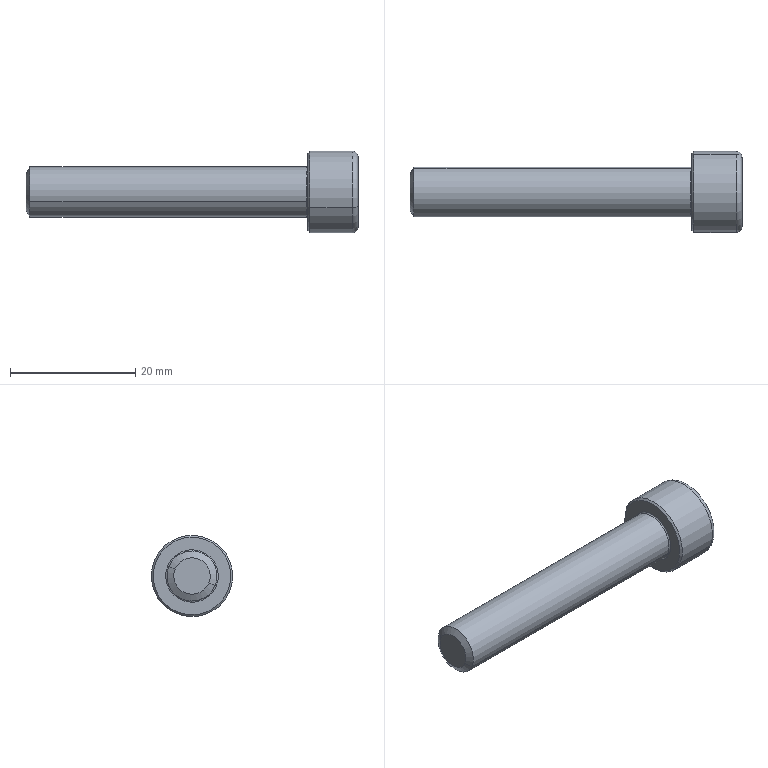Component | SolidWorks | M8_45_T70.1-1 | 1 solid | 28 faces | box 53 x 13 x 13 mm | volume 3185 mm3 | cone 10 | plane 10 | torus 4 | cylinder 4 | commonest cylinder face diameters 13 x2 8 x2 | material Plain Carbon Steel
STEP:
#1=COLOUR_RGB('',0.7922,0.8196,0.9333);
#2=FILL_AREA_STYLE_COLOUR('',#1);
#3=FILL_AREA_STYLE('',(#2));
#4=SURFACE_STYLE_FILL_AREA(#3);
#5=SURFACE_SIDE_STYLE('',(#4));
#6=SURFACE_STYLE_USAGE(.BOTH.,#5);
#7=PRESENTATION_STYLE_ASSIGNMENT((#6));
#8=CARTESIAN_POINT('',(2.524,1.896,1.764));
#9=VERTEX_POINT('',#8);
#10=CARTESIAN_POINT('',(2.524,1.445,1.577));
#11=VERTEX_POINT('',#10);
#12=CARTESIAN_POINT('',(2.524,1.67,1.67));
#13=DIRECTION('',(-1.,0.,-0.));
#14=DIRECTION('',(0.,-0.9242,-0.3818));
#15=AXIS2_PLACEMENT_3D('',#12,#13,#14);
#16=CIRCLE('',#15,0.2441);
#17=EDGE_CURVE('',#9,#11,#16,.T.);
#18=ORIENTED_EDGE('',*,*,#17,.F.);
#19=CARTESIAN_POINT('',(2.535,1.907,1.768));
#20=VERTEX_POINT('',#19);
#21=CARTESIAN_POINT('',(2.535,1.907,1.768));
#22=DIRECTION('',(0.7071,0.6535,0.27));
#23=VECTOR('',#22,39.37);
#24=LINE('',#21,#23);
#25=EDGE_CURVE('',#9,#20,#24,.T.);
#26=ORIENTED_EDGE('',*,*,#25,.T.);
#27=CARTESIAN_POINT('',(2.535,1.434,1.573));
#28=VERTEX_POINT('',#27);
#29=CARTESIAN_POINT('',(2.535,1.67,1.67));
#30=DIRECTION('',(1.,0.,0.));
#31=DIRECTION('',(0.,-0.9242,-0.3818));
#32=AXIS2_PLACEMENT_3D('',#29,#30,#31);
#33=CIRCLE('',#32,0.2559);
#34=EDGE_CURVE('',#28,#20,#33,.T.);
#35=ORIENTED_EDGE('',*,*,#34,.F.);
#36=CARTESIAN_POINT('',(2.535,1.434,1.573));
#37=DIRECTION('',(0.7071,-0.6535,-0.27));
#38=VECTOR('',#37,39.37);
#39=LINE('',#36,#38);
#40=EDGE_CURVE('',#11,#28,#39,.T.);
#41=ORIENTED_EDGE('',*,*,#40,.F.);
#42=EDGE_LOOP('',(#18,#26,#35,#41));
#43=FACE_OUTER_BOUND('',#42,.T.);
#44=CARTESIAN_POINT('',(2.535,1.67,1.67));
#45=DIRECTION('',(1.,0.,0.));
#46=DIRECTION('',(0.,-0.9242,-0.3818));
#47=AXIS2_PLACEMENT_3D('',#44,#45,#46);
#48=CONICAL_SURFACE('',#47,0.2559,0.7854);
#49=ADVANCED_FACE('',(#43),#48,.T.);
#50=CARTESIAN_POINT('',(2.839,1.467,1.586));
#51=VERTEX_POINT('',#50);
#52=CARTESIAN_POINT('',(2.839,1.874,1.755));
#53=VERTEX_POINT('',#52);
#54=CARTESIAN_POINT('',(2.839,1.67,1.67));
#55=DIRECTION('',(1.,0.,0.));
#56=DIRECTION('',(0.,0.9242,0.3818));
#57=AXIS2_PLACEMENT_3D('',#54,#55,#56);
#58=CIRCLE('',#57,0.2205);
#59=EDGE_CURVE('',#51,#53,#58,.T.);
#60=ORIENTED_EDGE('',*,*,#59,.F.);
#61=CARTESIAN_POINT('',(2.803,1.434,1.573));
#62=VERTEX_POINT('',#61);
#63=CARTESIAN_POINT('',(2.803,1.467,1.586));
#64=DIRECTION('',(0.,0.3818,-0.9242));
#65=DIRECTION('',(0.,0.9242,0.3818));
#66=AXIS2_PLACEMENT_3D('',#63,#64,#65);
#67=CIRCLE('',#66,0.03543);
#68=EDGE_CURVE('',#51,#62,#67,.T.);
#69=ORIENTED_EDGE('',*,*,#68,.T.);
#70=CARTESIAN_POINT('',(2.803,1.907,1.768));
#71=VERTEX_POINT('',#70);
#72=CARTESIAN_POINT('',(2.803,1.67,1.67));
#73=DIRECTION('',(-1.,0.,-0.));
#74=DIRECTION('',(0.,0.9242,0.3818));
#75=AXIS2_PLACEMENT_3D('',#72,#73,#74);
#76=CIRCLE('',#75,0.2559);
#77=EDGE_CURVE('',#71,#62,#76,.T.);
#78=ORIENTED_EDGE('',*,*,#77,.F.);
#79=CARTESIAN_POINT('',(2.803,1.874,1.755));
#80=DIRECTION('',(-0.,-0.3818,0.9242));
#81=DIRECTION('',(0.,-0.9242,-0.3818));
#82=AXIS2_PLACEMENT_3D('',#79,#80,#81);
#83=CIRCLE('',#82,0.03543);
#84=EDGE_CURVE('',#53,#71,#83,.T.);
#85=ORIENTED_EDGE('',*,*,#84,.F.);
#86=EDGE_LOOP('',(#60,#69,#78,#85));
#87=FACE_OUTER_BOUND('',#86,.T.);
#88=CARTESIAN_POINT('',(2.803,1.67,1.67));
#89=DIRECTION('',(-1.,0.,-0.));
#90=DIRECTION('',(-0.,0.9242,0.3818));
#91=AXIS2_PLACEMENT_3D('',#88,#89,#90);
#92=TOROIDAL_SURFACE('',#91,0.2205,0.03543);
#93=ADVANCED_FACE('',(#87),#92,.T.);
#94=CARTESIAN_POINT('',(0.752,1.564,1.626));
#95=VERTEX_POINT('',#94);
#96=CARTESIAN_POINT('',(0.752,1.776,1.714));
#97=VERTEX_POINT('',#96);
#98=CARTESIAN_POINT('',(0.752,1.67,1.67));
#99=DIRECTION('',(1.,0.,0.));
#100=DIRECTION('',(0.,-0.9242,-0.3818));
#101=AXIS2_PLACEMENT_3D('',#98,#99,#100);
#102=CIRCLE('',#101,0.1149);
#103=EDGE_CURVE('',#95,#97,#102,.T.);
#104=ORIENTED_EDGE('',*,*,#103,.T.);
#105=CARTESIAN_POINT('',(0.7766,1.816,1.73));
#106=VERTEX_POINT('',#105);
#107=CARTESIAN_POINT('',(0.7766,1.816,1.73));
#108=DIRECTION('',(0.5,0.8004,0.3307));
#109=VECTOR('',#108,39.37);
#110=LINE('',#107,#109);
#111=EDGE_CURVE('',#97,#106,#110,.T.);
#112=ORIENTED_EDGE('',*,*,#111,.T.);
#113=CARTESIAN_POINT('',(0.7766,1.525,1.61));
#114=VERTEX_POINT('',#113);
#115=CARTESIAN_POINT('',(0.7766,1.67,1.67));
#116=DIRECTION('',(1.,0.,0.));
#117=DIRECTION('',(0.,-0.9242,-0.3818));
#118=AXIS2_PLACEMENT_3D('',#115,#116,#117);
#119=CIRCLE('',#118,0.1575);
#120=EDGE_CURVE('',#114,#106,#119,.T.);
#121=ORIENTED_EDGE('',*,*,#120,.F.);
#122=CARTESIAN_POINT('',(0.7766,1.525,1.61));
#123=DIRECTION('',(0.5,-0.8004,-0.3307));
#124=VECTOR('',#123,39.37);
#125=LINE('',#122,#124);
#126=EDGE_CURVE('',#95,#114,#125,.T.);
#127=ORIENTED_EDGE('',*,*,#126,.F.);
#128=EDGE_LOOP('',(#104,#112,#121,#127));
#129=FACE_OUTER_BOUND('',#128,.T.);
#130=CARTESIAN_POINT('',(0.7766,1.67,1.67));
#131=DIRECTION('',(1.,0.,0.));
#132=DIRECTION('',(0.,-0.9242,-0.3818));
#133=AXIS2_PLACEMENT_3D('',#130,#131,#132);
#134=CONICAL_SURFACE('',#133,0.1575,1.047);
#135=ADVANCED_FACE('',(#129),#134,.T.);
#136=CARTESIAN_POINT('',(2.524,1.823,1.733));
#137=VERTEX_POINT('',#136);
#138=CARTESIAN_POINT('',(2.524,1.518,1.607));
#139=VERTEX_POINT('',#138);
#140=CARTESIAN_POINT('',(2.524,1.67,1.67));
#141=DIRECTION('',(1.,0.,0.));
#142=DIRECTION('',(0.,-0.9242,-0.3818));
#143=AXIS2_PLACEMENT_3D('',#140,#141,#142);
#144=CIRCLE('',#143,0.1654);
#145=EDGE_CURVE('',#137,#139,#144,.T.);
#146=ORIENTED_EDGE('',*,*,#145,.F.);
#147=CARTESIAN_POINT('',(2.516,1.816,1.73));
#148=VERTEX_POINT('',#147);
#149=CARTESIAN_POINT('',(2.516,1.823,1.733));
#150=DIRECTION('',(0.,0.3818,-0.9242));
#151=DIRECTION('',(0.,0.9242,0.3818));
#152=AXIS2_PLACEMENT_3D('',#149,#150,#151);
#153=CIRCLE('',#152,0.007874);
#154=EDGE_CURVE('',#137,#148,#153,.T.);
#155=ORIENTED_EDGE('',*,*,#154,.T.);
#156=CARTESIAN_POINT('',(2.516,1.525,1.61));
#157=VERTEX_POINT('',#156);
#158=CARTESIAN_POINT('',(2.516,1.67,1.67));
#159=DIRECTION('',(1.,0.,0.));
#160=DIRECTION('',(0.,-0.9242,-0.3818));
#161=AXIS2_PLACEMENT_3D('',#158,#159,#160);
#162=CIRCLE('',#161,0.1575);
#163=EDGE_CURVE('',#148,#157,#162,.T.);
#164=ORIENTED_EDGE('',*,*,#163,.T.);
#165=CARTESIAN_POINT('',(2.516,1.518,1.607));
#166=DIRECTION('',(-0.,-0.3818,0.9242));
#167=DIRECTION('',(0.,-0.9242,-0.3818));
#168=AXIS2_PLACEMENT_3D('',#165,#166,#167);
#169=CIRCLE('',#168,0.007874);
#170=EDGE_CURVE('',#139,#157,#169,.T.);
#171=ORIENTED_EDGE('',*,*,#170,.F.);
#172=EDGE_LOOP('',(#146,#155,#164,#171));
#173=FACE_OUTER_BOUND('',#172,.T.);
#174=CARTESIAN_POINT('',(2.516,1.67,1.67));
#175=DIRECTION('',(1.,0.,0.));
#176=DIRECTION('',(0.,-0.9242,-0.3818));
#177=AXIS2_PLACEMENT_3D('',#174,#175,#176);
#178=TOROIDAL_SURFACE('',#177,0.1654,0.007874);
#179=ADVANCED_FACE('',(#173),#178,.F.);
#180=ORIENTED_EDGE('',*,*,#34,.T.);
#181=CARTESIAN_POINT('',(2.839,1.907,1.768));
#182=DIRECTION('',(1.,0.,0.));
#183=VECTOR('',#182,39.37);
#184=LINE('',#181,#183);
#185=EDGE_CURVE('',#20,#71,#184,.T.);
#186=ORIENTED_EDGE('',*,*,#185,.T.);
#187=ORIENTED_EDGE('',*,*,#77,.T.);
#188=CARTESIAN_POINT('',(2.839,1.434,1.573));
#189=DIRECTION('',(1.,0.,0.));
#190=VECTOR('',#189,39.37);
#191=LINE('',#188,#190);
#192=EDGE_CURVE('',#28,#62,#191,.T.);
#193=ORIENTED_EDGE('',*,*,#192,.F.);
#194=EDGE_LOOP('',(#180,#186,#187,#193));
#195=FACE_OUTER_BOUND('',#194,.T.);
#196=CARTESIAN_POINT('',(2.839,1.67,1.67));
#197=DIRECTION('',(1.,0.,0.));
#198=DIRECTION('',(0.,-0.9242,-0.3818));
#199=AXIS2_PLACEMENT_3D('',#196,#197,#198);
#200=CYLINDRICAL_SURFACE('',#199,0.2559);
#201=ADVANCED_FACE('',(#195),#200,.T.);
#202=ORIENTED_EDGE('',*,*,#120,.T.);
#203=CARTESIAN_POINT('',(2.839,1.816,1.73));
#204=DIRECTION('',(1.,0.,0.));
#205=VECTOR('',#204,39.37);
#206=LINE('',#203,#205);
#207=EDGE_CURVE('',#106,#148,#206,.T.);
#208=ORIENTED_EDGE('',*,*,#207,.T.);
#209=CARTESIAN_POINT('',(2.516,1.67,1.67));
#210=DIRECTION('',(1.,0.,0.));
#211=DIRECTION('',(0.,-0.9242,-0.3818));
#212=AXIS2_PLACEMENT_3D('',#209,#210,#211);
#213=CIRCLE('',#212,0.1575);
#214=EDGE_CURVE('',#157,#148,#213,.T.);
#215=ORIENTED_EDGE('',*,*,#214,.F.);
#216=CARTESIAN_POINT('',(2.839,1.525,1.61));
#217=DIRECTION('',(1.,0.,0.));
#218=VECTOR('',#217,39.37);
#219=LINE('',#216,#218);
#220=EDGE_CURVE('',#114,#157,#219,.T.);
#221=ORIENTED_EDGE('',*,*,#220,.F.);
#222=EDGE_LOOP('',(#202,#208,#215,#221));
#223=FACE_OUTER_BOUND('',#222,.T.);
#224=CARTESIAN_POINT('',(2.839,1.67,1.67));
#225=DIRECTION('',(1.,0.,0.));
#226=DIRECTION('',(0.,-0.9242,-0.3818));
#227=AXIS2_PLACEMENT_3D('',#224,#225,#226);
#228=CYLINDRICAL_SURFACE('',#227,0.1575);
#229=ADVANCED_FACE('',(#223),#228,.T.);
#230=ORIENTED_EDGE('',*,*,#207,.F.);
#231=CARTESIAN_POINT('',(0.7766,1.67,1.67));
#232=DIRECTION('',(1.,0.,0.));
#233=DIRECTION('',(0.,-0.9242,-0.3818));
#234=AXIS2_PLACEMENT_3D('',#231,#232,#233);
#235=CIRCLE('',#234,0.1575);
#236=EDGE_CURVE('',#106,#114,#235,.T.);
#237=ORIENTED_EDGE('',*,*,#236,.T.);
#238=ORIENTED_EDGE('',*,*,#220,.T.);
#239=ORIENTED_EDGE('',*,*,#163,.F.);
#240=EDGE_LOOP('',(#230,#237,#238,#239));
#241=FACE_OUTER_BOUND('',#240,.T.);
#242=CARTESIAN_POINT('',(2.839,1.67,1.67));
#243=DIRECTION('',(1.,0.,0.));
#244=DIRECTION('',(0.,-0.9242,-0.3818));
#245=AXIS2_PLACEMENT_3D('',#242,#243,#244);
#246=CYLINDRICAL_SURFACE('',#245,0.1575);
#247=ADVANCED_FACE('',(#241),#246,.T.);
#248=CARTESIAN_POINT('',(2.839,1.67,1.67));
#249=DIRECTION('',(1.,0.,0.));
#250=DIRECTION('',(0.,0.9242,0.3818));
#251=AXIS2_PLACEMENT_3D('',#248,#249,#250);
#252=CIRCLE('',#251,0.2205);
#253=EDGE_CURVE('',#53,#51,#252,.T.);
#254=ORIENTED_EDGE('',*,*,#253,.T.);
#255=ORIENTED_EDGE('',*,*,#59,.T.);
#256=EDGE_LOOP('',(#254,#255));
#257=FACE_OUTER_BOUND('',#256,.T.);
#258=CARTESIAN_POINT('',(2.839,1.795,1.722));
#259=VERTEX_POINT('',#258);
#260=CARTESIAN_POINT('',(2.839,1.688,1.804));
#261=VERTEX_POINT('',#260);
#262=CARTESIAN_POINT('',(2.839,1.67,1.67));
#263=DIRECTION('',(1.,0.,0.));
#264=DIRECTION('',(0.,-0.9242,-0.3818));
#265=AXIS2_PLACEMENT_3D('',#262,#263,#264);
#266=CIRCLE('',#265,0.135);
#267=EDGE_CURVE('',#259,#261,#266,.T.);
#268=ORIENTED_EDGE('',*,*,#267,.F.);
#269=CARTESIAN_POINT('',(2.839,1.777,1.588));
#270=VERTEX_POINT('',#269);
#271=CARTESIAN_POINT('',(2.839,1.67,1.67));
#272=DIRECTION('',(1.,0.,0.));
#273=DIRECTION('',(0.,-0.9242,-0.3818));
#274=AXIS2_PLACEMENT_3D('',#271,#272,#273);
#275=CIRCLE('',#274,0.135);
#276=EDGE_CURVE('',#270,#259,#275,.T.);
#277=ORIENTED_EDGE('',*,*,#276,.F.);
#278=CARTESIAN_POINT('',(2.839,1.653,1.536));
#279=VERTEX_POINT('',#278);
#280=CARTESIAN_POINT('',(2.839,1.67,1.67));
#281=DIRECTION('',(1.,0.,0.));
#282=DIRECTION('',(0.,-0.9242,-0.3818));
#283=AXIS2_PLACEMENT_3D('',#280,#281,#282);
#284=CIRCLE('',#283,0.135);
#285=EDGE_CURVE('',#279,#270,#284,.T.);
#286=ORIENTED_EDGE('',*,*,#285,.F.);
#287=CARTESIAN_POINT('',(2.839,1.546,1.619));
#288=VERTEX_POINT('',#287);
#289=CARTESIAN_POINT('',(2.839,1.67,1.67));
#290=DIRECTION('',(1.,0.,0.));
#291=DIRECTION('',(0.,-0.9242,-0.3818));
#292=AXIS2_PLACEMENT_3D('',#289,#290,#291);
#293=CIRCLE('',#292,0.135);
#294=EDGE_CURVE('',#288,#279,#293,.T.);
#295=ORIENTED_EDGE('',*,*,#294,.F.);
#296=CARTESIAN_POINT('',(2.839,1.563,1.753));
#297=VERTEX_POINT('',#296);
#298=CARTESIAN_POINT('',(2.839,1.67,1.67));
#299=DIRECTION('',(1.,0.,0.));
#300=DIRECTION('',(0.,-0.9242,-0.3818));
#301=AXIS2_PLACEMENT_3D('',#298,#299,#300);
#302=CIRCLE('',#301,0.135);
#303=EDGE_CURVE('',#297,#288,#302,.T.);
#304=ORIENTED_EDGE('',*,*,#303,.F.);
#305=CARTESIAN_POINT('',(2.839,1.67,1.67));
#306=DIRECTION('',(1.,0.,0.));
#307=DIRECTION('',(0.,-0.9242,-0.3818));
#308=AXIS2_PLACEMENT_3D('',#305,#306,#307);
#309=CIRCLE('',#308,0.135);
#310=EDGE_CURVE('',#261,#297,#309,.T.);
#311=ORIENTED_EDGE('',*,*,#310,.F.);
#312=EDGE_LOOP('',(#268,#277,#286,#295,#304,#311));
#313=FACE_BOUND('',#312,.T.);
#314=CARTESIAN_POINT('',(2.839,1.67,1.67));
#315=DIRECTION('',(-1.,0.,-0.));
#316=DIRECTION('',(-0.,0.9242,0.3818));
#317=AXIS2_PLACEMENT_3D('',#314,#315,#316);
#318=PLANE('',#317);
#319=ADVANCED_FACE('',(#257,#313),#318,.F.);
#320=ORIENTED_EDGE('',*,*,#185,.F.);
#321=CARTESIAN_POINT('',(2.535,1.67,1.67));
#322=DIRECTION('',(1.,0.,0.));
#323=DIRECTION('',(0.,-0.9242,-0.3818));
#324=AXIS2_PLACEMENT_3D('',#321,#322,#323);
#325=CIRCLE('',#324,0.2559);
#326=EDGE_CURVE('',#20,#28,#325,.T.);
#327=ORIENTED_EDGE('',*,*,#326,.T.);
#328=ORIENTED_EDGE('',*,*,#192,.T.);
#329=CARTESIAN_POINT('',(2.803,1.67,1.67));
#330=DIRECTION('',(-1.,0.,-0.));
#331=DIRECTION('',(0.,0.9242,0.3818));
#332=AXIS2_PLACEMENT_3D('',#329,#330,#331);
#333=CIRCLE('',#332,0.2559);
#334=EDGE_CURVE('',#62,#71,#333,.T.);
#335=ORIENTED_EDGE('',*,*,#334,.T.);
#336=EDGE_LOOP('',(#320,#327,#328,#335));
#337=FACE_OUTER_BOUND('',#336,.T.);
#338=CARTESIAN_POINT('',(2.839,1.67,1.67));
#339=DIRECTION('',(1.,0.,0.));
#340=DIRECTION('',(0.,-0.9242,-0.3818));
#341=AXIS2_PLACEMENT_3D('',#338,#339,#340);
#342=CYLINDRICAL_SURFACE('',#341,0.2559);
#343=ADVANCED_FACE('',(#337),#342,.T.);
#344=CARTESIAN_POINT('',(2.524,1.67,1.67));
#345=DIRECTION('',(-1.,0.,-0.));
#346=DIRECTION('',(0.,-0.9242,-0.3818));
#347=AXIS2_PLACEMENT_3D('',#344,#345,#346);
#348=CIRCLE('',#347,0.2441);
#349=EDGE_CURVE('',#11,#9,#348,.T.);
#350=ORIENTED_EDGE('',*,*,#349,.T.);
#351=ORIENTED_EDGE('',*,*,#17,.T.);
#352=EDGE_LOOP('',(#350,#351));
#353=FACE_OUTER_BOUND('',#352,.T.);
#354=CARTESIAN_POINT('',(2.524,1.67,1.67));
#355=DIRECTION('',(1.,0.,0.));
#356=DIRECTION('',(0.,-0.9242,-0.3818));
#357=AXIS2_PLACEMENT_3D('',#354,#355,#356);
#358=CIRCLE('',#357,0.1654);
#359=EDGE_CURVE('',#139,#137,#358,.T.);
#360=ORIENTED_EDGE('',*,*,#359,.T.);
#361=ORIENTED_EDGE('',*,*,#145,.T.);
#362=EDGE_LOOP('',(#360,#361));
#363=FACE_BOUND('',#362,.T.);
#364=CARTESIAN_POINT('',(2.524,1.768,1.434));
#365=DIRECTION('',(1.,-0.,0.));
#366=DIRECTION('',(0.,-0.9242,-0.3818));
#367=AXIS2_PLACEMENT_3D('',#364,#365,#366);
#368=PLANE('',#367);
#369=ADVANCED_FACE('',(#353,#363),#368,.F.);
#370=ORIENTED_EDGE('',*,*,#154,.F.);
#371=ORIENTED_EDGE('',*,*,#359,.F.);
#372=ORIENTED_EDGE('',*,*,#170,.T.);
#373=ORIENTED_EDGE('',*,*,#214,.T.);
#374=EDGE_LOOP('',(#370,#371,#372,#373));
#375=FACE_OUTER_BOUND('',#374,.T.);
#376=CARTESIAN_POINT('',(2.516,1.67,1.67));
#377=DIRECTION('',(1.,0.,0.));
#378=DIRECTION('',(0.,-0.9242,-0.3818));
#379=AXIS2_PLACEMENT_3D('',#376,#377,#378);
#380=TOROIDAL_SURFACE('',#379,0.1654,0.007874);
#381=ADVANCED_FACE('',(#375),#380,.F.);
#382=ORIENTED_EDGE('',*,*,#111,.F.);
#383=CARTESIAN_POINT('',(0.752,1.67,1.67));
#384=DIRECTION('',(1.,0.,0.));
#385=DIRECTION('',(0.,-0.9242,-0.3818));
#386=AXIS2_PLACEMENT_3D('',#383,#384,#385);
#387=CIRCLE('',#386,0.1149);
#388=EDGE_CURVE('',#97,#95,#387,.T.);
#389=ORIENTED_EDGE('',*,*,#388,.T.);
#390=ORIENTED_EDGE('',*,*,#126,.T.);
#391=ORIENTED_EDGE('',*,*,#236,.F.);
#392=EDGE_LOOP('',(#382,#389,#390,#391));
#393=FACE_OUTER_BOUND('',#392,.T.);
#394=CARTESIAN_POINT('',(0.7766,1.67,1.67));
#395=DIRECTION('',(1.,0.,0.));
#396=DIRECTION('',(0.,-0.9242,-0.3818));
#397=AXIS2_PLACEMENT_3D('',#394,#395,#396);
#398=CONICAL_SURFACE('',#397,0.1575,1.047);
#399=ADVANCED_FACE('',(#393),#398,.T.);
#400=ORIENTED_EDGE('',*,*,#103,.F.);
#401=ORIENTED_EDGE('',*,*,#388,.F.);
#402=EDGE_LOOP('',(#400,#401));
#403=FACE_OUTER_BOUND('',#402,.T.);
#404=CARTESIAN_POINT('',(0.752,1.73,1.525));
#405=DIRECTION('',(1.,-0.,0.));
#406=DIRECTION('',(0.,-0.9242,-0.3818));
#407=AXIS2_PLACEMENT_3D('',#404,#405,#406);
#408=PLANE('',#407);
#409=ADVANCED_FACE('',(#403),#408,.F.);
#410=ORIENTED_EDGE('',*,*,#68,.F.);
#411=ORIENTED_EDGE('',*,*,#253,.F.);
#412=ORIENTED_EDGE('',*,*,#84,.T.);
#413=ORIENTED_EDGE('',*,*,#334,.F.);
#414=EDGE_LOOP('',(#410,#411,#412,#413));
#415=FACE_OUTER_BOUND('',#414,.T.);
#416=CARTESIAN_POINT('',(2.803,1.67,1.67));
#417=DIRECTION('',(-1.,0.,-0.));
#418=DIRECTION('',(-0.,0.9242,0.3818));
#419=AXIS2_PLACEMENT_3D('',#416,#417,#418);
#420=TOROIDAL_SURFACE('',#419,0.2205,0.03543);
#421=ADVANCED_FACE('',(#415),#420,.T.);
#422=ORIENTED_EDGE('',*,*,#25,.F.);
#423=ORIENTED_EDGE('',*,*,#349,.F.);
#424=ORIENTED_EDGE('',*,*,#40,.T.);
#425=ORIENTED_EDGE('',*,*,#326,.F.);
#426=EDGE_LOOP('',(#422,#423,#424,#425));
#427=FACE_OUTER_BOUND('',#426,.T.);
#428=CARTESIAN_POINT('',(2.535,1.67,1.67));
#429=DIRECTION('',(1.,0.,0.));
#430=DIRECTION('',(0.,-0.9242,-0.3818));
#431=AXIS2_PLACEMENT_3D('',#428,#429,#430);
#432=CONICAL_SURFACE('',#431,0.2559,0.7854);
#433=ADVANCED_FACE('',(#427),#432,.T.);
#434=ORIENTED_EDGE('',*,*,#294,.T.);
#435=CARTESIAN_POINT('',(2.839,1.546,1.619));
#436=CARTESIAN_POINT('',(2.832,1.563,1.605));
#437=CARTESIAN_POINT('',(2.828,1.581,1.592));
#438=CARTESIAN_POINT('',(2.828,1.608,1.571));
#439=CARTESIAN_POINT('',(2.829,1.617,1.564));
#440=CARTESIAN_POINT('',(2.833,1.635,1.55));
#441=CARTESIAN_POINT('',(2.835,1.644,1.543));
#442=CARTESIAN_POINT('',(2.839,1.653,1.536));
#443=B_SPLINE_CURVE_WITH_KNOTS('',3,(#435,#436,#437,#438,#439,#440,#441,#442),.UNSPECIFIED.,.F.,.F.,(4,2,2,4),(0.00000024,0.001732,0.002598,0.003464),.UNSPECIFIED.);
#444=EDGE_CURVE('',#288,#279,#443,.T.);
#445=ORIENTED_EDGE('',*,*,#444,.F.);
#446=EDGE_LOOP('',(#434,#445));
#447=FACE_OUTER_BOUND('',#446,.T.);
#448=CARTESIAN_POINT('',(2.839,1.67,1.67));
#449=DIRECTION('',(1.,0.,0.));
#450=DIRECTION('',(0.,-0.9242,-0.3818));
#451=AXIS2_PLACEMENT_3D('',#448,#449,#450);
#452=CONICAL_SURFACE('',#451,0.135,1.047);
#453=ADVANCED_FACE('',(#447),#452,.F.);
#454=ORIENTED_EDGE('',*,*,#285,.T.);
#455=CARTESIAN_POINT('',(2.839,1.653,1.536));
#456=CARTESIAN_POINT('',(2.835,1.663,1.541));
#457=CARTESIAN_POINT('',(2.833,1.673,1.545));
#458=CARTESIAN_POINT('',(2.829,1.694,1.553));
#459=CARTESIAN_POINT('',(2.828,1.704,1.558));
#460=CARTESIAN_POINT('',(2.828,1.726,1.567));
#461=CARTESIAN_POINT('',(2.829,1.736,1.571));
#462=CARTESIAN_POINT('',(2.833,1.757,1.58));
#463=CARTESIAN_POINT('',(2.835,1.767,1.584));
#464=CARTESIAN_POINT('',(2.839,1.777,1.588));
#465=B_SPLINE_CURVE_WITH_KNOTS('',3,(#455,#456,#457,#458,#459,#460,#461,#462,#463,#464),.UNSPECIFIED.,.F.,.F.,(4,2,2,2,4),(0.009185,0.01005,0.01092,0.01179,0.01266),.UNSPECIFIED.);
#466=EDGE_CURVE('',#279,#270,#465,.T.);
#467=ORIENTED_EDGE('',*,*,#466,.F.);
#468=EDGE_LOOP('',(#454,#467));
#469=FACE_OUTER_BOUND('',#468,.T.);
#470=CARTESIAN_POINT('',(2.839,1.67,1.67));
#471=DIRECTION('',(1.,0.,0.));
#472=DIRECTION('',(0.,-0.9242,-0.3818));
#473=AXIS2_PLACEMENT_3D('',#470,#471,#472);
#474=CONICAL_SURFACE('',#473,0.135,1.047);
#475=ADVANCED_FACE('',(#469),#474,.F.);
#476=ORIENTED_EDGE('',*,*,#276,.T.);
#477=CARTESIAN_POINT('',(2.839,1.777,1.588));
#478=CARTESIAN_POINT('',(2.832,1.78,1.61));
#479=CARTESIAN_POINT('',(2.828,1.783,1.632));
#480=CARTESIAN_POINT('',(2.828,1.788,1.666));
#481=CARTESIAN_POINT('',(2.829,1.789,1.678));
#482=CARTESIAN_POINT('',(2.833,1.792,1.7));
#483=CARTESIAN_POINT('',(2.835,1.794,1.711));
#484=CARTESIAN_POINT('',(2.839,1.795,1.722));
#485=B_SPLINE_CURVE_WITH_KNOTS('',3,(#477,#478,#479,#480,#481,#482,#483,#484),.UNSPECIFIED.,.F.,.F.,(4,2,2,4),(0.00000024,0.001732,0.002598,0.003464),.UNSPECIFIED.);
#486=EDGE_CURVE('',#270,#259,#485,.T.);
#487=ORIENTED_EDGE('',*,*,#486,.F.);
#488=EDGE_LOOP('',(#476,#487));
#489=FACE_OUTER_BOUND('',#488,.T.);
#490=CARTESIAN_POINT('',(2.839,1.67,1.67));
#491=DIRECTION('',(1.,0.,0.));
#492=DIRECTION('',(0.,-0.9242,-0.3818));
#493=AXIS2_PLACEMENT_3D('',#490,#491,#492);
#494=CONICAL_SURFACE('',#493,0.135,1.047);
#495=ADVANCED_FACE('',(#489),#494,.F.);
#496=ORIENTED_EDGE('',*,*,#267,.T.);
#497=CARTESIAN_POINT('',(2.839,1.795,1.722));
#498=CARTESIAN_POINT('',(2.832,1.778,1.735));
#499=CARTESIAN_POINT('',(2.828,1.76,1.749));
#500=CARTESIAN_POINT('',(2.828,1.733,1.77));
#501=CARTESIAN_POINT('',(2.829,1.724,1.777));
#502=CARTESIAN_POINT('',(2.833,1.706,1.791));
#503=CARTESIAN_POINT('',(2.835,1.697,1.797));
#504=CARTESIAN_POINT('',(2.839,1.688,1.804));
#505=B_SPLINE_CURVE_WITH_KNOTS('',3,(#497,#498,#499,#500,#501,#502,#503,#504),.UNSPECIFIED.,.F.,.F.,(4,2,2,4),(0.00000024,0.001732,0.002598,0.003464),.UNSPECIFIED.);
#506=EDGE_CURVE('',#259,#261,#505,.T.);
#507=ORIENTED_EDGE('',*,*,#506,.F.);
#508=EDGE_LOOP('',(#496,#507));
#509=FACE_OUTER_BOUND('',#508,.T.);
#510=CARTESIAN_POINT('',(2.839,1.67,1.67));
#511=DIRECTION('',(1.,0.,0.));
#512=DIRECTION('',(0.,-0.9242,-0.3818));
#513=AXIS2_PLACEMENT_3D('',#510,#511,#512);
#514=CONICAL_SURFACE('',#513,0.135,1.047);
#515=ADVANCED_FACE('',(#509),#514,.F.);
#516=ORIENTED_EDGE('',*,*,#310,.T.);
#517=CARTESIAN_POINT('',(2.839,1.688,1.804));
#518=CARTESIAN_POINT('',(2.835,1.678,1.8));
#519=CARTESIAN_POINT('',(2.833,1.668,1.796));
#520=CARTESIAN_POINT('',(2.829,1.647,1.787));
#521=CARTESIAN_POINT('',(2.828,1.636,1.783));
#522=CARTESIAN_POINT('',(2.828,1.615,1.774));
#523=CARTESIAN_POINT('',(2.829,1.604,1.77));
#524=CARTESIAN_POINT('',(2.833,1.584,1.761));
#525=CARTESIAN_POINT('',(2.835,1.573,1.757));
#526=CARTESIAN_POINT('',(2.839,1.563,1.753));
#527=B_SPLINE_CURVE_WITH_KNOTS('',3,(#517,#518,#519,#520,#521,#522,#523,#524,#525,#526),.UNSPECIFIED.,.F.,.F.,(4,2,2,2,4),(0.002941,0.003808,0.004675,0.005542,0.006409),.UNSPECIFIED.);
#528=EDGE_CURVE('',#261,#297,#527,.T.);
#529=ORIENTED_EDGE('',*,*,#528,.F.);
#530=EDGE_LOOP('',(#516,#529));
#531=FACE_OUTER_BOUND('',#530,.T.);
#532=CARTESIAN_POINT('',(2.839,1.67,1.67));
#533=DIRECTION('',(1.,0.,0.));
#534=DIRECTION('',(0.,-0.9242,-0.3818));
#535=AXIS2_PLACEMENT_3D('',#532,#533,#534);
#536=CONICAL_SURFACE('',#535,0.135,1.047);
#537=ADVANCED_FACE('',(#531),#536,.F.);
#538=ORIENTED_EDGE('',*,*,#303,.T.);
#539=CARTESIAN_POINT('',(2.839,1.563,1.753));
#540=CARTESIAN_POINT('',(2.832,1.56,1.731));
#541=CARTESIAN_POINT('',(2.828,1.557,1.709));
#542=CARTESIAN_POINT('',(2.828,1.553,1.674));
#543=CARTESIAN_POINT('',(2.829,1.551,1.663));
#544=CARTESIAN_POINT('',(2.833,1.548,1.641));
#545=CARTESIAN_POINT('',(2.835,1.547,1.63));
#546=CARTESIAN_POINT('',(2.839,1.546,1.619));
#547=B_SPLINE_CURVE_WITH_KNOTS('',3,(#539,#540,#541,#542,#543,#544,#545,#546),.UNSPECIFIED.,.F.,.F.,(4,2,2,4),(0.00000024,0.001732,0.002598,0.003464),.UNSPECIFIED.);
#548=EDGE_CURVE('',#297,#288,#547,.T.);
#549=ORIENTED_EDGE('',*,*,#548,.F.);
#550=EDGE_LOOP('',(#538,#549));
#551=FACE_OUTER_BOUND('',#550,.T.);
#552=CARTESIAN_POINT('',(2.839,1.67,1.67));
#553=DIRECTION('',(1.,0.,0.));
#554=DIRECTION('',(0.,-0.9242,-0.3818));
#555=AXIS2_PLACEMENT_3D('',#552,#553,#554);
#556=CONICAL_SURFACE('',#555,0.135,1.047);
#557=ADVANCED_FACE('',(#551),#556,.F.);
#558=CARTESIAN_POINT('',(2.681,1.563,1.753));
#559=VERTEX_POINT('',#558);
#560=CARTESIAN_POINT('',(2.681,1.546,1.619));
#561=VERTEX_POINT('',#560);
#562=CARTESIAN_POINT('',(2.681,1.563,1.753));
#563=DIRECTION('',(0.,-0.1314,-0.9913));
#564=VECTOR('',#563,39.37);
#565=LINE('',#562,#564);
#566=EDGE_CURVE('',#559,#561,#565,.T.);
#567=ORIENTED_EDGE('',*,*,#566,.T.);
#568=CARTESIAN_POINT('',(2.681,1.653,1.536));
#569=VERTEX_POINT('',#568);
#570=CARTESIAN_POINT('',(2.681,1.546,1.619));
#571=DIRECTION('',(0.,0.7928,-0.6095));
#572=VECTOR('',#571,39.37);
#573=LINE('',#570,#572);
#574=EDGE_CURVE('',#561,#569,#573,.T.);
#575=ORIENTED_EDGE('',*,*,#574,.T.);
#576=CARTESIAN_POINT('',(2.681,1.777,1.588));
#577=VERTEX_POINT('',#576);
#578=CARTESIAN_POINT('',(2.681,1.653,1.536));
#579=DIRECTION('',(-0.,0.9242,0.3818));
#580=VECTOR('',#579,39.37);
#581=LINE('',#578,#580);
#582=EDGE_CURVE('',#569,#577,#581,.T.);
#583=ORIENTED_EDGE('',*,*,#582,.T.);
#584=CARTESIAN_POINT('',(2.681,1.795,1.722));
#585=VERTEX_POINT('',#584);
#586=CARTESIAN_POINT('',(2.681,1.777,1.588));
#587=DIRECTION('',(-0.,0.1314,0.9913));
#588=VECTOR('',#587,39.37);
#589=LINE('',#586,#588);
#590=EDGE_CURVE('',#577,#585,#589,.T.);
#591=ORIENTED_EDGE('',*,*,#590,.T.);
#592=CARTESIAN_POINT('',(2.681,1.688,1.804));
#593=VERTEX_POINT('',#592);
#594=CARTESIAN_POINT('',(2.681,1.795,1.722));
#595=DIRECTION('',(-0.,-0.7928,0.6095));
#596=VECTOR('',#595,39.37);
#597=LINE('',#594,#596);
#598=EDGE_CURVE('',#585,#593,#597,.T.);
#599=ORIENTED_EDGE('',*,*,#598,.T.);
#600=CARTESIAN_POINT('',(2.681,1.688,1.804));
#601=DIRECTION('',(0.,-0.9242,-0.3818));
#602=VECTOR('',#601,39.37);
#603=LINE('',#600,#602);
#604=EDGE_CURVE('',#593,#559,#603,.T.);
#605=ORIENTED_EDGE('',*,*,#604,.T.);
#606=EDGE_LOOP('',(#567,#575,#583,#591,#599,#605));
#607=FACE_OUTER_BOUND('',#606,.T.);
#608=CARTESIAN_POINT('',(2.681,1.563,1.753));
#609=DIRECTION('',(-1.,0.,-0.));
#610=DIRECTION('',(-0.,0.9242,0.3818));
#611=AXIS2_PLACEMENT_3D('',#608,#609,#610);
#612=PLANE('',#611);
#613=ADVANCED_FACE('',(#607),#612,.F.);
#614=CARTESIAN_POINT('',(2.681,1.546,1.619));
#615=DIRECTION('',(1.,0.,0.));
#616=VECTOR('',#615,39.37);
#617=LINE('',#614,#616);
#618=EDGE_CURVE('',#561,#288,#617,.T.);
#619=ORIENTED_EDGE('',*,*,#618,.T.);
#620=ORIENTED_EDGE('',*,*,#444,.T.);
#621=CARTESIAN_POINT('',(2.681,1.653,1.536));
#622=DIRECTION('',(1.,0.,0.));
#623=VECTOR('',#622,39.37);
#624=LINE('',#621,#623);
#625=EDGE_CURVE('',#569,#279,#624,.T.);
#626=ORIENTED_EDGE('',*,*,#625,.F.);
#627=ORIENTED_EDGE('',*,*,#574,.F.);
#628=EDGE_LOOP('',(#619,#620,#626,#627));
#629=FACE_OUTER_BOUND('',#628,.T.);
#630=CARTESIAN_POINT('',(2.681,1.546,1.619));
#631=DIRECTION('',(0.,-0.6095,-0.7928));
#632=DIRECTION('',(-0.,-0.7928,0.6095));
#633=AXIS2_PLACEMENT_3D('',#630,#631,#632);
#634=PLANE('',#633);
#635=ADVANCED_FACE('',(#629),#634,.F.);
#636=ORIENTED_EDGE('',*,*,#625,.T.);
#637=ORIENTED_EDGE('',*,*,#466,.T.);
#638=CARTESIAN_POINT('',(2.681,1.777,1.588));
#639=DIRECTION('',(1.,0.,0.));
#640=VECTOR('',#639,39.37);
#641=LINE('',#638,#640);
#642=EDGE_CURVE('',#577,#270,#641,.T.);
#643=ORIENTED_EDGE('',*,*,#642,.F.);
#644=ORIENTED_EDGE('',*,*,#582,.F.);
#645=EDGE_LOOP('',(#636,#637,#643,#644));
#646=FACE_OUTER_BOUND('',#645,.T.);
#647=CARTESIAN_POINT('',(2.681,1.653,1.536));
#648=DIRECTION('',(0.,0.3818,-0.9242));
#649=DIRECTION('',(0.,-0.9242,-0.3818));
#650=AXIS2_PLACEMENT_3D('',#647,#648,#649);
#651=PLANE('',#650);
#652=ADVANCED_FACE('',(#646),#651,.F.);
#653=ORIENTED_EDGE('',*,*,#642,.T.);
#654=ORIENTED_EDGE('',*,*,#486,.T.);
#655=CARTESIAN_POINT('',(2.681,1.795,1.722));
#656=DIRECTION('',(1.,0.,0.));
#657=VECTOR('',#656,39.37);
#658=LINE('',#655,#657);
#659=EDGE_CURVE('',#585,#259,#658,.T.);
#660=ORIENTED_EDGE('',*,*,#659,.F.);
#661=ORIENTED_EDGE('',*,*,#590,.F.);
#662=EDGE_LOOP('',(#653,#654,#660,#661));
#663=FACE_OUTER_BOUND('',#662,.T.);
#664=CARTESIAN_POINT('',(2.681,1.777,1.588));
#665=DIRECTION('',(0.,0.9913,-0.1314));
#666=DIRECTION('',(0.,-0.1314,-0.9913));
#667=AXIS2_PLACEMENT_3D('',#664,#665,#666);
#668=PLANE('',#667);
#669=ADVANCED_FACE('',(#663),#668,.F.);
#670=ORIENTED_EDGE('',*,*,#659,.T.);
#671=ORIENTED_EDGE('',*,*,#506,.T.);
#672=CARTESIAN_POINT('',(2.681,1.688,1.804));
#673=DIRECTION('',(1.,0.,0.));
#674=VECTOR('',#673,39.37);
#675=LINE('',#672,#674);
#676=EDGE_CURVE('',#593,#261,#675,.T.);
#677=ORIENTED_EDGE('',*,*,#676,.F.);
#678=ORIENTED_EDGE('',*,*,#598,.F.);
#679=EDGE_LOOP('',(#670,#671,#677,#678));
#680=FACE_OUTER_BOUND('',#679,.T.);
#681=CARTESIAN_POINT('',(2.681,1.795,1.722));
#682=DIRECTION('',(-0.,0.6095,0.7928));
#683=DIRECTION('',(0.,0.7928,-0.6095));
#684=AXIS2_PLACEMENT_3D('',#681,#682,#683);
#685=PLANE('',#684);
#686=ADVANCED_FACE('',(#680),#685,.F.);
#687=ORIENTED_EDGE('',*,*,#676,.T.);
#688=ORIENTED_EDGE('',*,*,#528,.T.);
#689=CARTESIAN_POINT('',(2.681,1.563,1.753));
#690=DIRECTION('',(1.,0.,0.));
#691=VECTOR('',#690,39.37);
#692=LINE('',#689,#691);
#693=EDGE_CURVE('',#559,#297,#692,.T.);
#694=ORIENTED_EDGE('',*,*,#693,.F.);
#695=ORIENTED_EDGE('',*,*,#604,.F.);
#696=EDGE_LOOP('',(#687,#688,#694,#695));
#697=FACE_OUTER_BOUND('',#696,.T.);
#698=CARTESIAN_POINT('',(2.681,1.688,1.804));
#699=DIRECTION('',(-0.,-0.3818,0.9242));
#700=DIRECTION('',(-0.,0.9242,0.3818));
#701=AXIS2_PLACEMENT_3D('',#698,#699,#700);
#702=PLANE('',#701);
#703=ADVANCED_FACE('',(#697),#702,.F.);
#704=ORIENTED_EDGE('',*,*,#693,.T.);
#705=ORIENTED_EDGE('',*,*,#548,.T.);
#706=ORIENTED_EDGE('',*,*,#618,.F.);
#707=ORIENTED_EDGE('',*,*,#566,.F.);
#708=EDGE_LOOP('',(#704,#705,#706,#707));
#709=FACE_OUTER_BOUND('',#708,.T.);
#710=CARTESIAN_POINT('',(2.681,1.563,1.753));
#711=DIRECTION('',(-0.,-0.9913,0.1314));
#712=DIRECTION('',(-0.,0.1314,0.9913));
#713=AXIS2_PLACEMENT_3D('',#710,#711,#712);
#714=PLANE('',#713);
#715=ADVANCED_FACE('',(#709),#714,.F.);
#716=CLOSED_SHELL('',(#49,#93,#135,#179,#201,#229,#247,#319,#343,#369,#381,#399,#409,#421,#433,#453,#475,#495,#515,#537,#557,#613,#635,#652,#669,#686,#703,#715));
#717=MANIFOLD_SOLID_BREP('',#716);
#718=STYLED_ITEM('',(#7),#717);
#719=PRESENTATION_LAYER_ASSIGNMENT('','',(#718));
#720=(LENGTH_UNIT()NAMED_UNIT(*)SI_UNIT($,.METRE.));
#721=LENGTH_MEASURE_WITH_UNIT(LENGTH_MEASURE(0.0254),#720);
#722=DIMENSIONAL_EXPONENTS(1.,0.,0.,0.,0.,0.,0.);
#723=(CONVERSION_BASED_UNIT('',#721)LENGTH_UNIT()NAMED_UNIT(#722));
#724=UNCERTAINTY_MEASURE_WITH_UNIT(LENGTH_MEASURE(0.00001),#723,'','');
#725=(NAMED_UNIT(*)PLANE_ANGLE_UNIT()SI_UNIT($,.RADIAN.));
#726=(NAMED_UNIT(*)SI_UNIT($,.STERADIAN.)SOLID_ANGLE_UNIT());
#727=(GEOMETRIC_REPRESENTATION_CONTEXT(3)GLOBAL_UNCERTAINTY_ASSIGNED_CONTEXT((#724))GLOBAL_UNIT_ASSIGNED_CONTEXT((#723,#725,#726))REPRESENTATION_CONTEXT('',''));
#728=MECHANICAL_DESIGN_GEOMETRIC_PRESENTATION_REPRESENTATION('',(#718),#727);
#729=CARTESIAN_POINT('',(0.,0.,0.));
#730=DIRECTION('',(0.,0.,1.));
#731=DIRECTION('',(1.,0.,0.));
#732=AXIS2_PLACEMENT_3D('',#729,#730,#731);
#733=(LENGTH_UNIT()NAMED_UNIT(*)SI_UNIT($,.METRE.));
#734=LENGTH_MEASURE_WITH_UNIT(LENGTH_MEASURE(0.0254),#733);
#735=DIMENSIONAL_EXPONENTS(1.,0.,0.,0.,0.,0.,0.);
#736=(CONVERSION_BASED_UNIT('',#734)LENGTH_UNIT()NAMED_UNIT(#735));
#737=UNCERTAINTY_MEASURE_WITH_UNIT(LENGTH_MEASURE(0.00001),#736,'','');
#738=(NAMED_UNIT(*)PLANE_ANGLE_UNIT()SI_UNIT($,.RADIAN.));
#739=(NAMED_UNIT(*)SI_UNIT($,.STERADIAN.)SOLID_ANGLE_UNIT());
#740=(GEOMETRIC_REPRESENTATION_CONTEXT(3)GLOBAL_UNCERTAINTY_ASSIGNED_CONTEXT((#737))GLOBAL_UNIT_ASSIGNED_CONTEXT((#736,#738,#739))REPRESENTATION_CONTEXT('',''));
#741=ADVANCED_BREP_SHAPE_REPRESENTATION('',(#717,#732),#740);